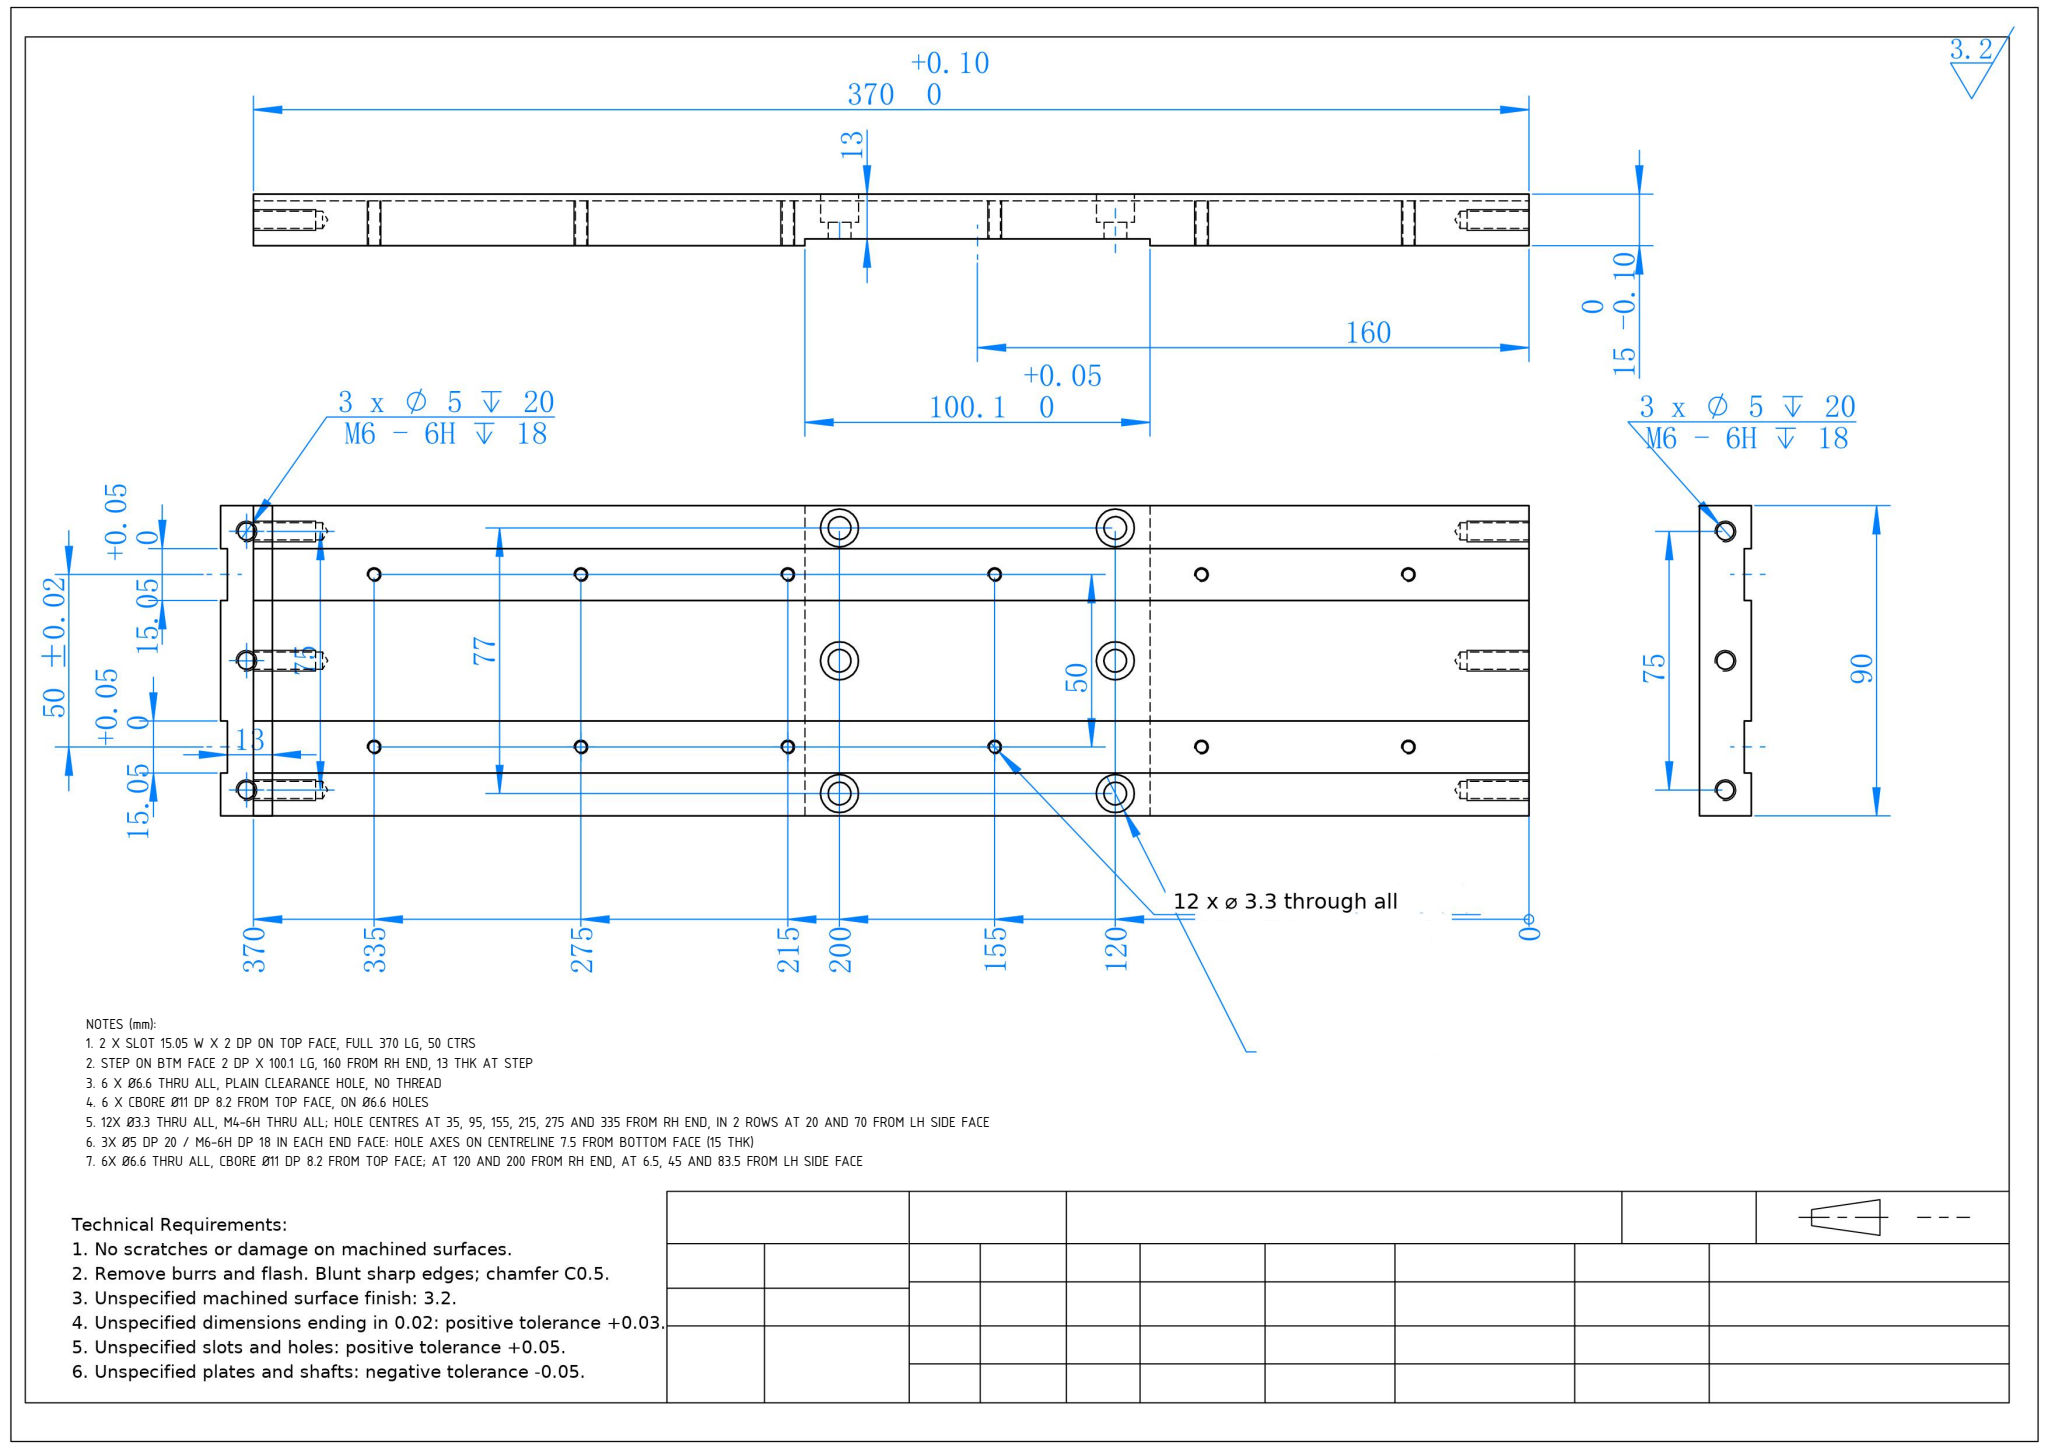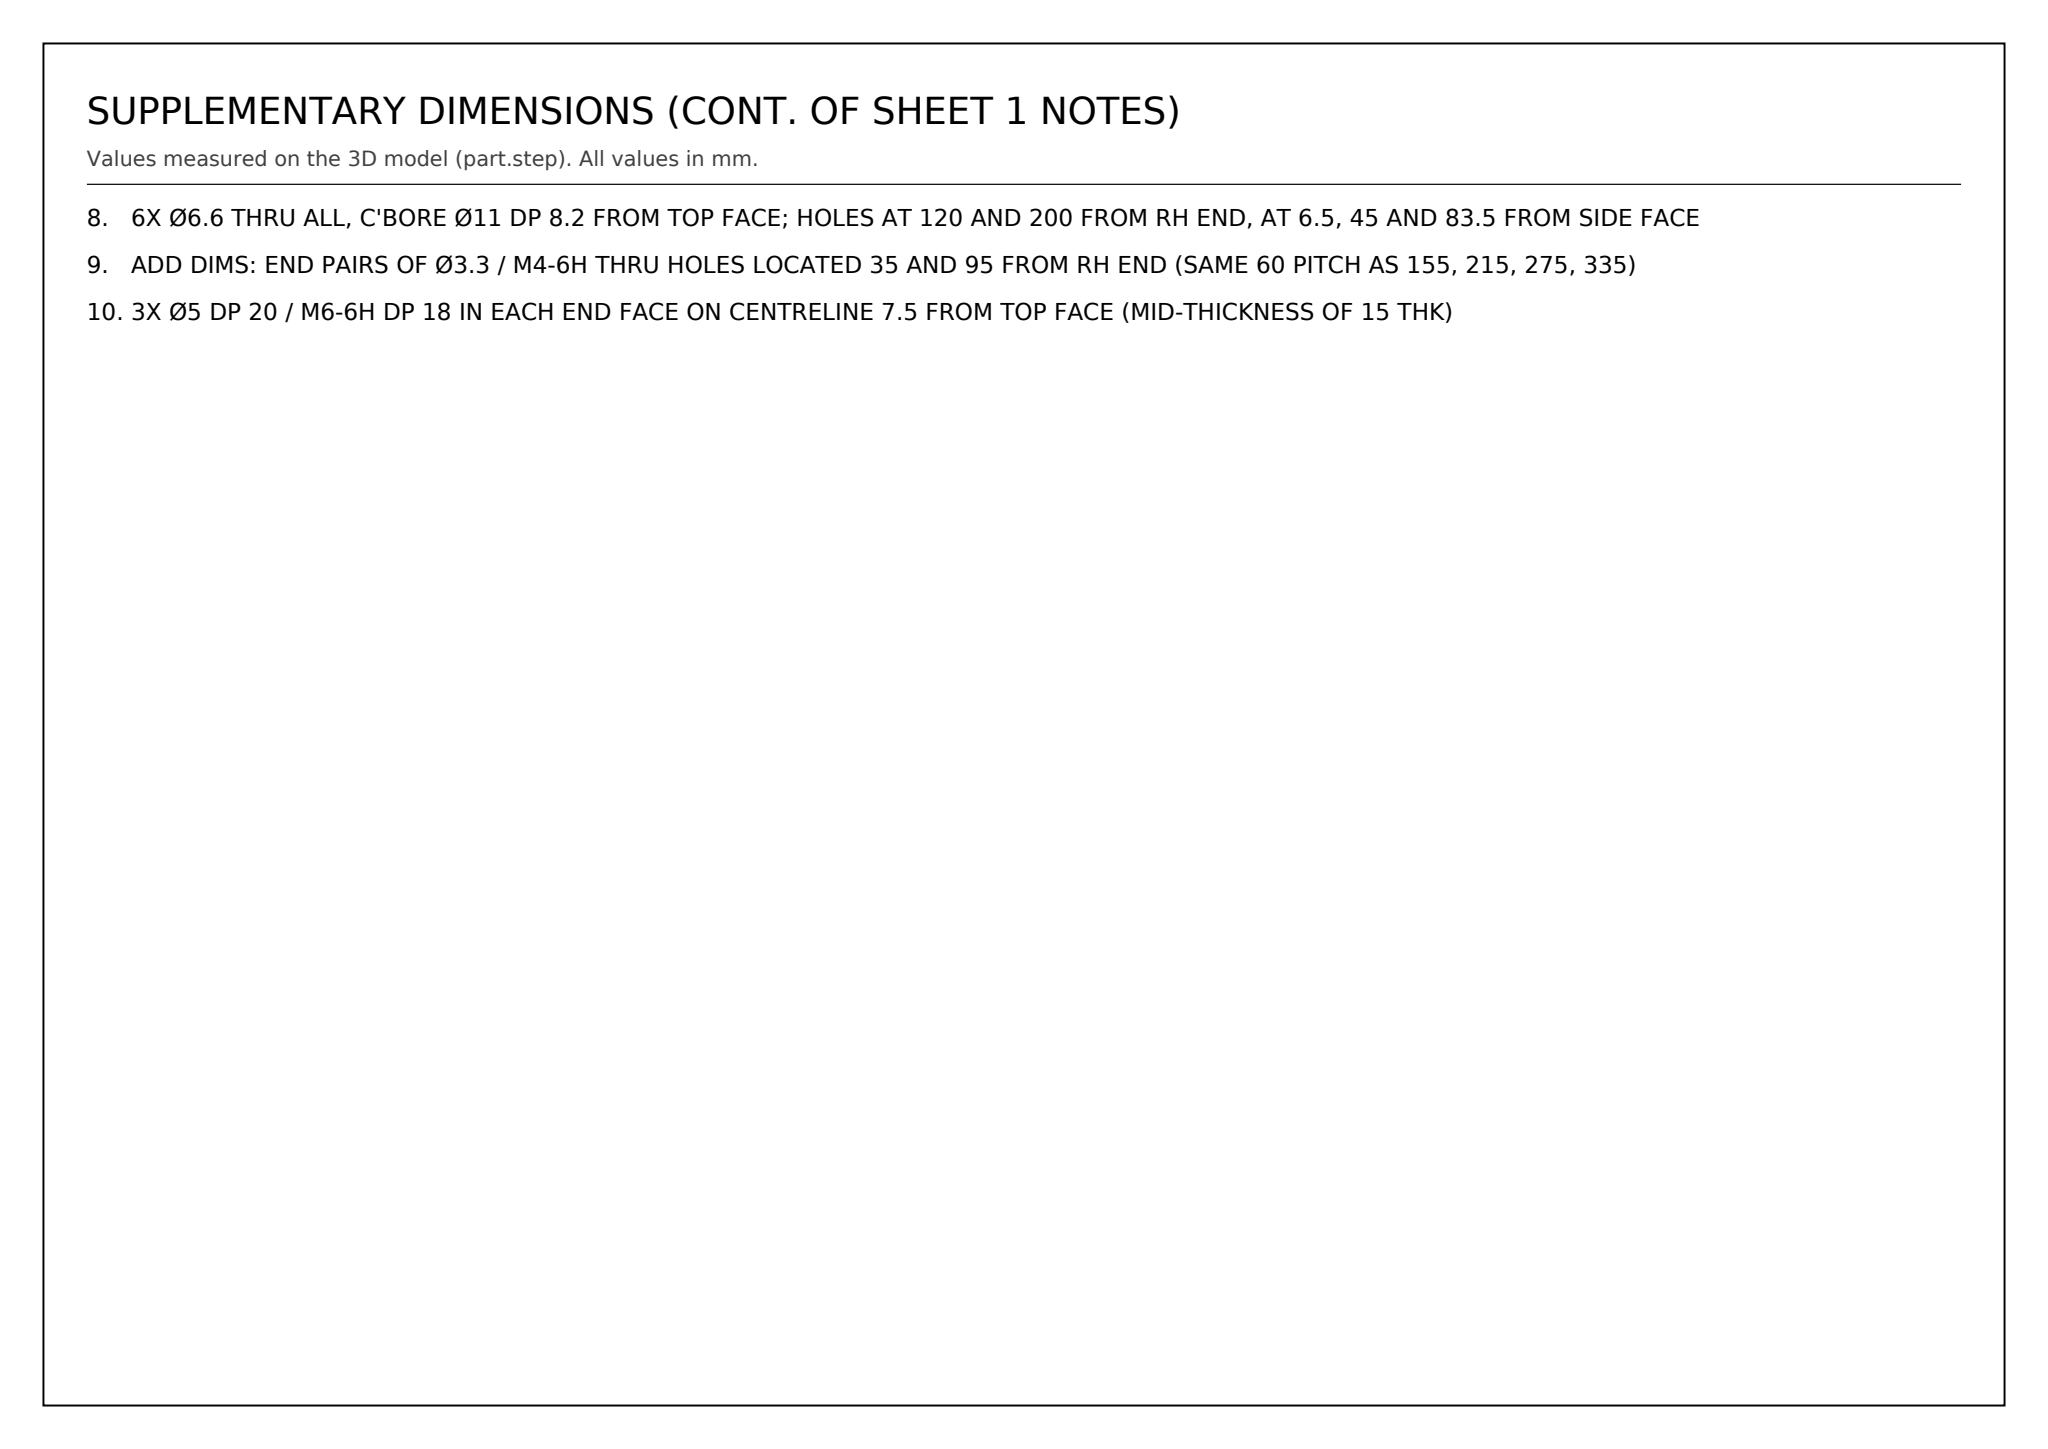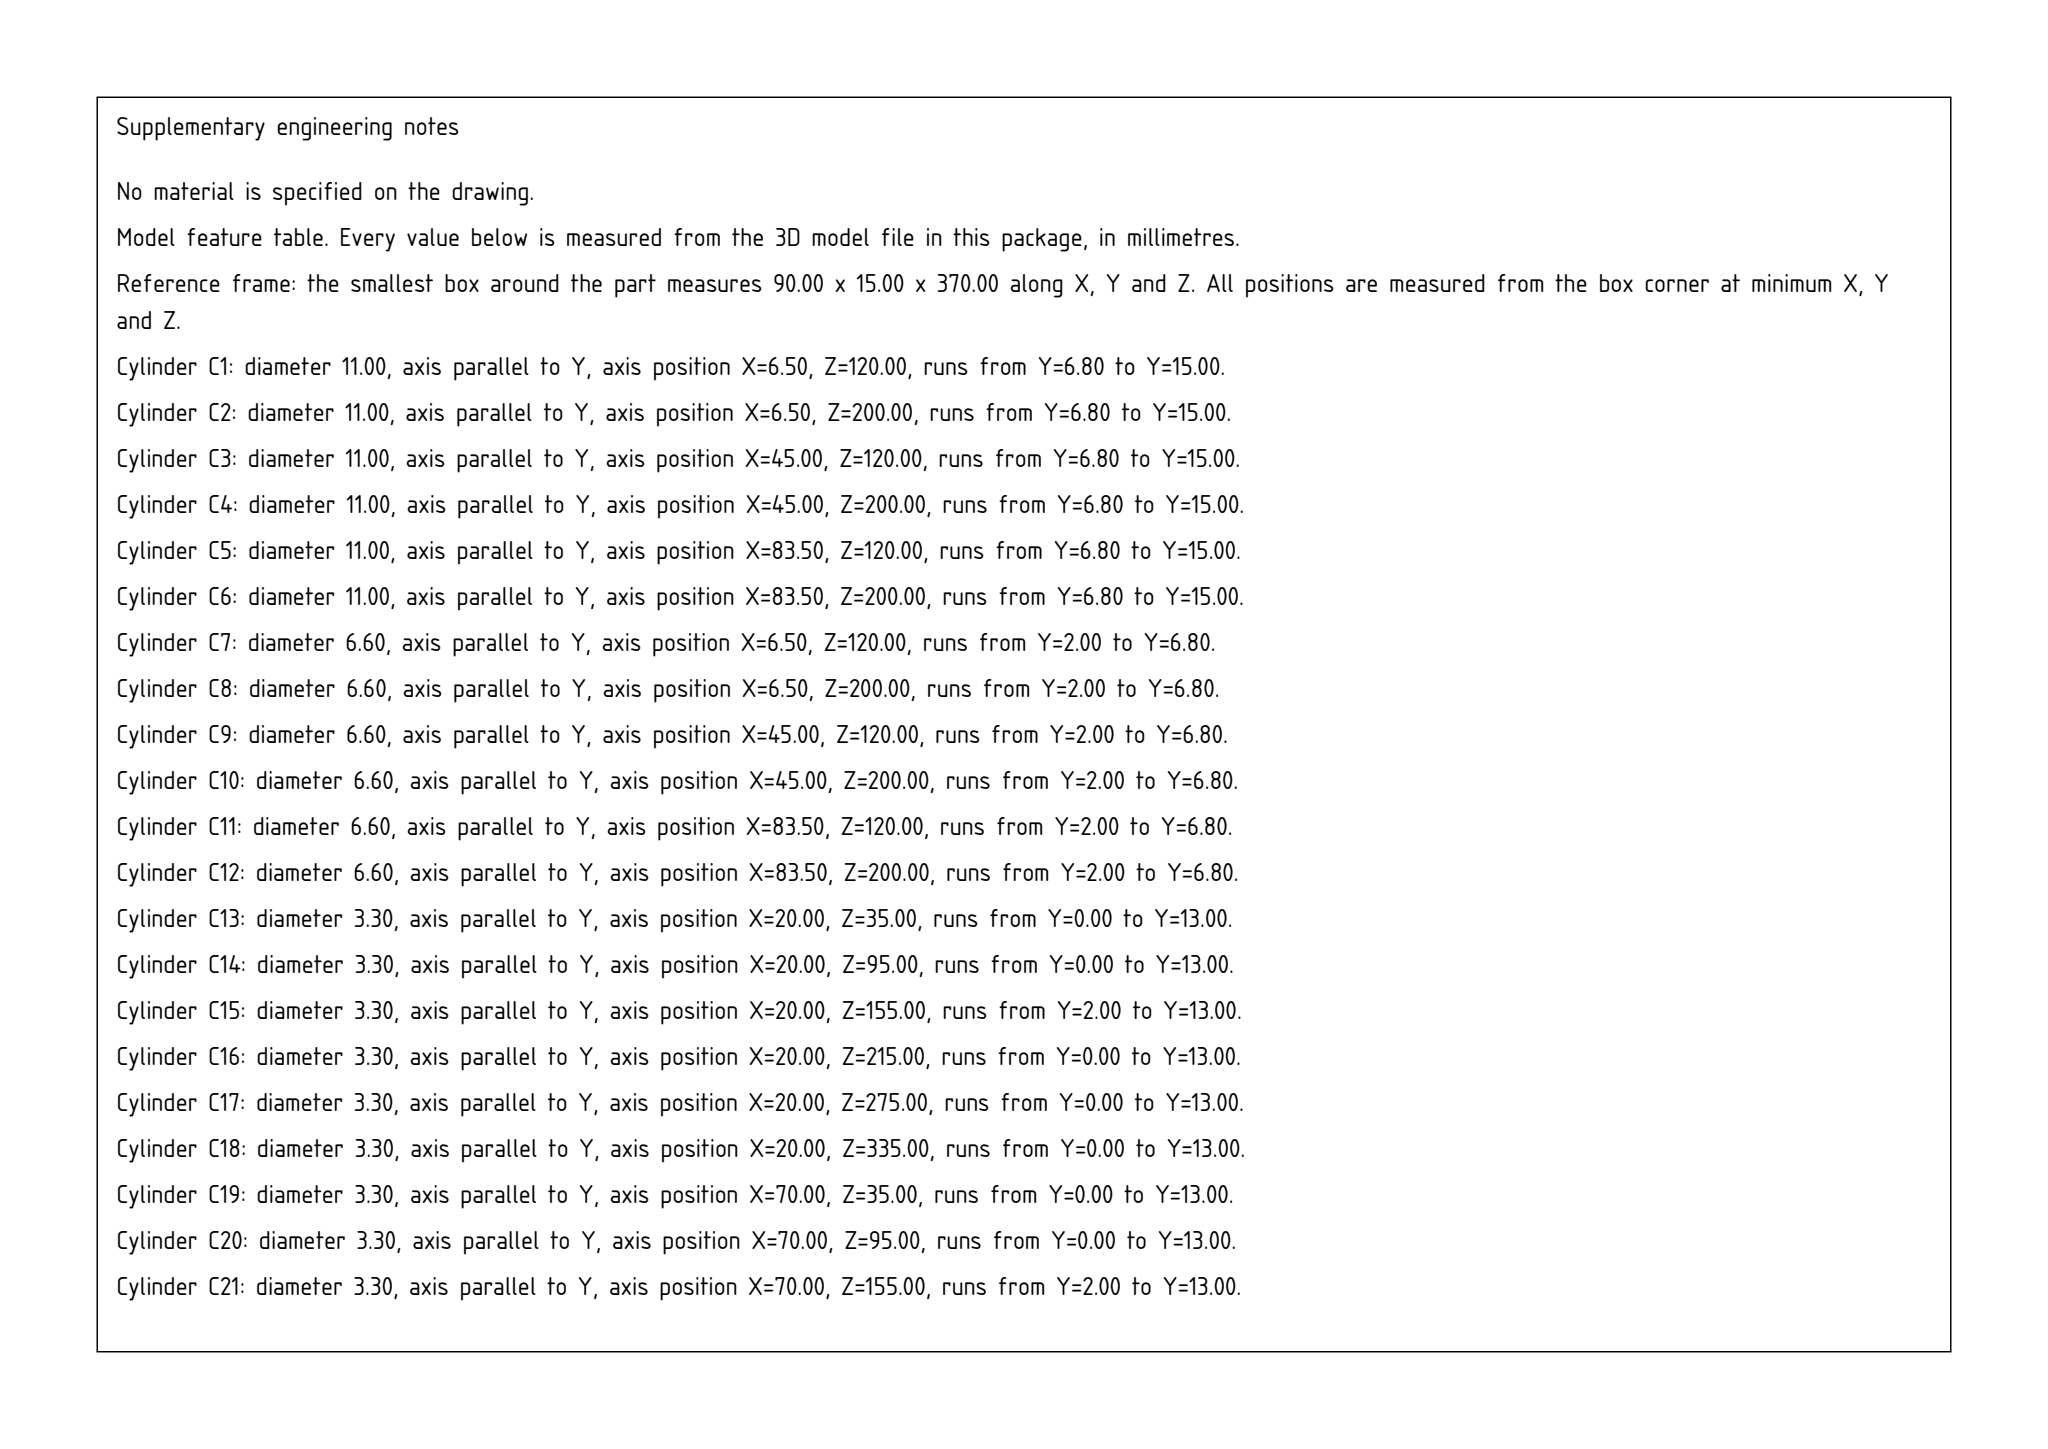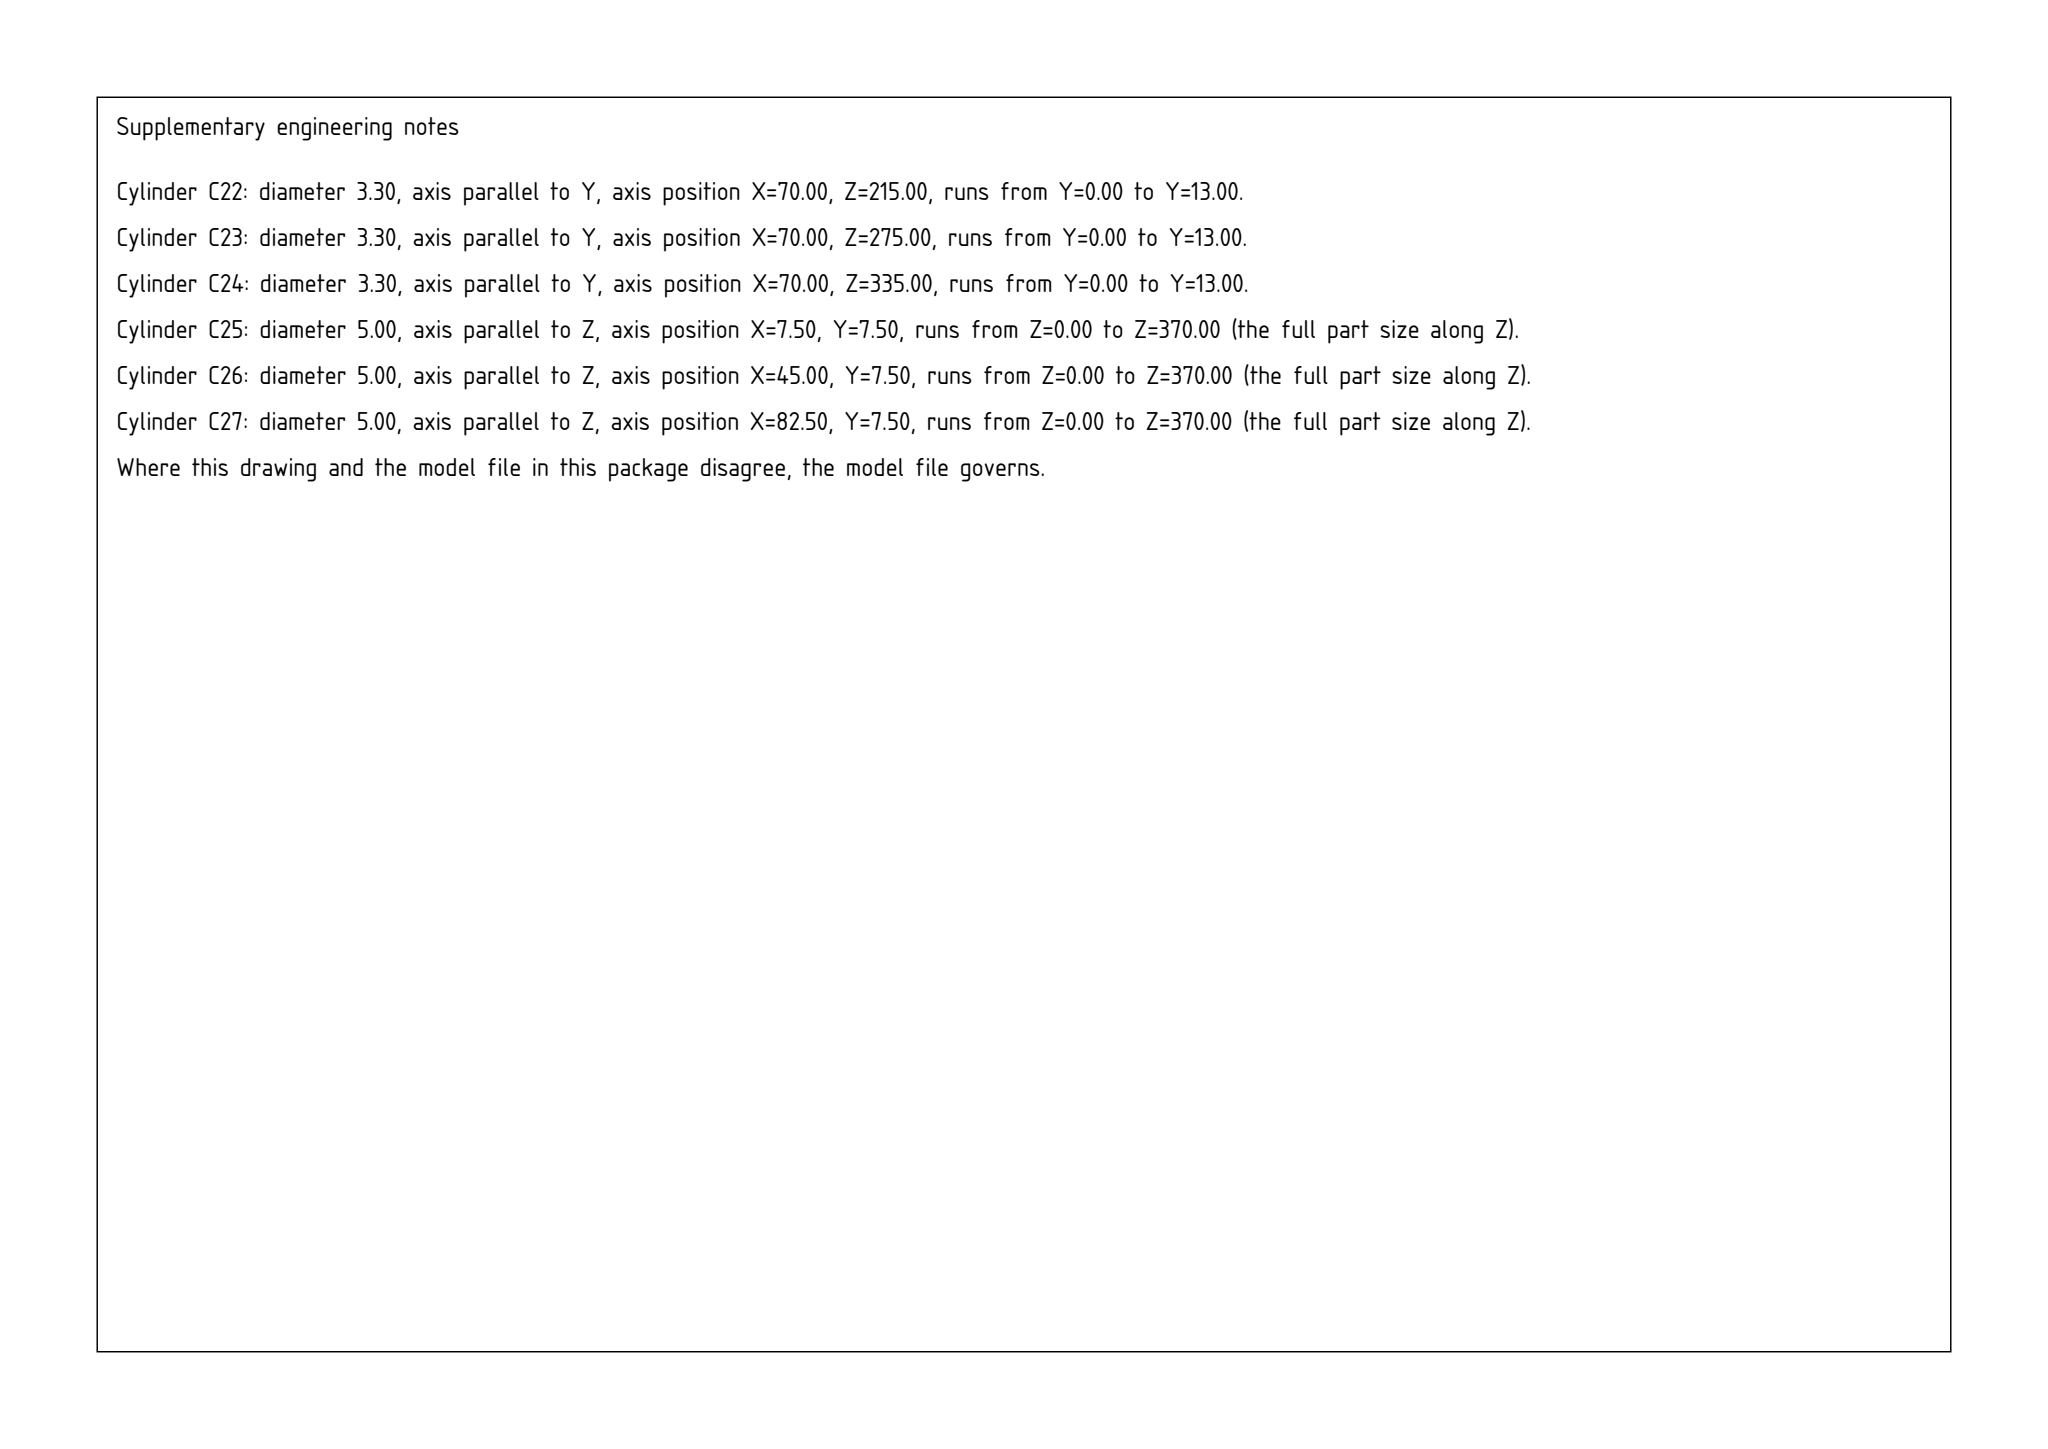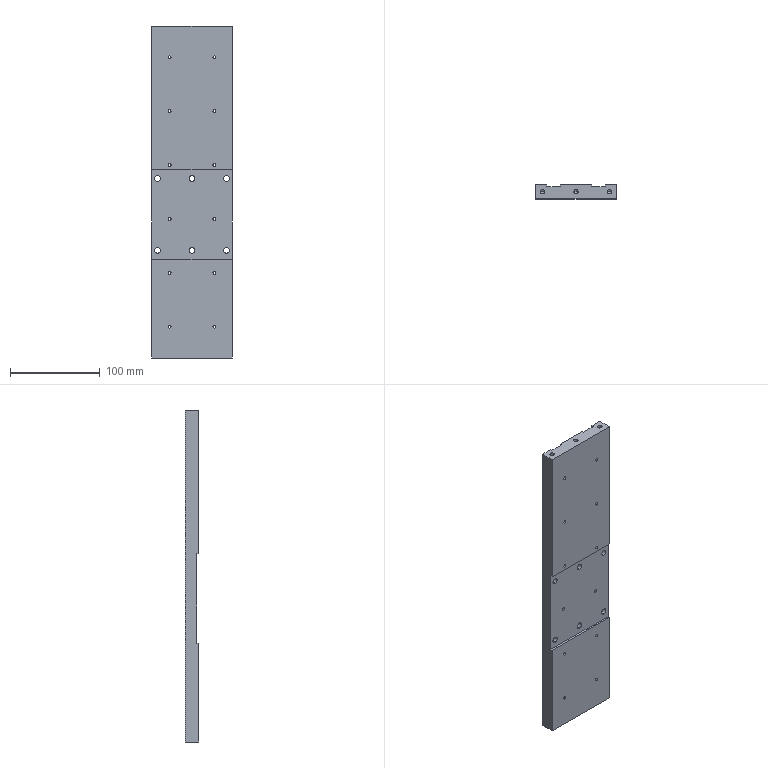Part | SolidWorks | mm | 1 solid | 96 faces | box 90 x 15 x 370 mm | volume 449832 mm3 | cylinder 60 | plane 24 | cone 12 | commonest cylinder face diameters 3.3 x24 11 x12 6.6 x12 5 x12
Drawing notes:
2 X SLOT 15.05 W X 2 DP ON TOP FACE, FULL 370 LG, 50 CTRS | from the solid: x planes 12.48/27.53 & 62.48/77.53 (w=15.05, CL 20.0 & 70.0); floor y=13 vs top y=15
STEP ON BTM FACE 2 DP X 100.1 LG, 160 FROM RH END, 13 THK AT STEP | from the solid: z planes 109.95 & 210.05 (100.1 lg), 370-210.05=160; floor y=2.0, thk 13
6 X Ø6.6 THRU ALL, PLAIN CLEARANCE HOLE, NO THREAD | from the solid: cyl Ø6.6 axis y len 4.8 at x=6.5/45/83.5, z=120 & 200 (6 plcs)
6 X CBORE Ø11 DP 8.2 FROM TOP FACE, ON Ø6.6 HOLES | from the solid: cyl Ø11 axis y len 8.2, floor y=6.8 (6 plcs) from top y=15
12X Ø3.3 THRU ALL, M4-6H THRU ALL; HOLE CENTRES AT 35, 95, 155, 215, 275 AND 335 FROM RH END, IN 2 ROWS AT 20 AND 70 FROM LH SIDE FACE | from the solid: cylinders dia 3.3 axis y at z=35, 95, 155, 215, 275, 335 and x=20.0 / 70.0
3X Ø5 DP 20 / M6-6H DP 18 IN EACH END FACE: HOLE AXES ON CENTRELINE 7.5 FROM BOTTOM FACE (15 THK) | from the solid: cylinders dia 5.0 axis z, pos_other_axes y=7.5, length 20.0
6X Ø6.6 THRU ALL, CBORE Ø11 DP 8.2 FROM TOP FACE; AT 120 AND 200 FROM RH END, AT 6.5, 45 AND 83.5 FROM LH SIDE FACE | from the solid: cylinders dia 6.6 (len 4.8) and dia 11.0 (len 8.2) axis y at z=120.0, 200.0 and x=6.5, 45.0, 83.5
6X Ø6.6 THRU ALL, C'BORE Ø11 DP 8.2 FROM TOP FACE; HOLES AT 120 AND 200 FROM RH END, AT 6.5, 45 AND 83.5 FROM SIDE FACE | from the solid: cylinders dia 6.6 axis y at (6.5/45/83.5, z=120 & 200) len 4.8 and dia 11.0 axis y same positions len 8.2
ADD DIMS: END PAIRS OF Ø3.3 / M4-6H THRU HOLES LOCATED 35 AND 95 FROM RH END (SAME 60 PITCH AS 155, 215, 275, 335) | from the solid: cylinders dia 3.3 axis y at z=35 and z=95, x=20.0 and 70.0
3X Ø5 DP 20 / M6-6H DP 18 IN EACH END FACE ON CENTRELINE 7.5 FROM TOP FACE (MID-THICKNESS OF 15 THK) | from the solid: cylinders dia 5.0 axis z at y=7.5 (x=7.5, 45.0, 82.5), length 20.0
build123d program:
from build123d import *

# Parameters (mm, degrees)
SKETCH1_W                                       = 90
SKETCH1_H                                       = 15
EXTRUDE1_DEPTH                                  = 185
SKETCH16_W                                      = 15.05
SKETCH16_H                                      = 370
CUT_EXTRUDE1_DEPTH                              = 2
SKETCH17_W                                      = 90
SKETCH17_H                                      = 100.1
CUT_EXTRUDE2_DEPTH                              = 2
M6_TAPPED_HOLE1_D                               = 5
M6_TAPPED_HOLE1_DEPTH                           = 20
M6_TAPPED_HOLE1_TIP                             = 1.502
M6_TAPPED_HOLE2_D                               = 5
M6_TAPPED_HOLE2_DEPTH                           = 20
M6_TAPPED_HOLE2_TIP                             = 1.502
M6_HEX_SOCKET_HEAD_CAP_SCREW_CBORE1_D           = 6.6
M6_HEX_SOCKET_HEAD_CAP_SCREW_CBORE1_CBORE_D     = 11
M6_HEX_SOCKET_HEAD_CAP_SCREW_CBORE1_CBORE_DEPTH = 8.2
M4_TAPPED_HOLE8_D                               = 3.3


with BuildPart() as part:
    # Sketch1 → Extrude1 (new, symmetric)
    with BuildSketch(Plane.XY):
        Rectangle(SKETCH1_W, SKETCH1_H)
    extrude(amount=EXTRUDE1_DEPTH, both=True)

    # Sketch16 → Cut-Extrude1 (cut)
    with BuildSketch(Plane(origin=(0, 7.5, 0), x_dir=(1, 0, 0), z_dir=(0, 1, 0))):
        with Locations((25, 0)):
            Rectangle(SKETCH16_W, SKETCH16_H)
        with Locations((-25, 0)):
            Rectangle(SKETCH16_W, SKETCH16_H)
    extrude(amount=-CUT_EXTRUDE1_DEPTH, mode=Mode.SUBTRACT)

    # Sketch17 → Cut-Extrude2 (cut)
    with BuildSketch(Plane(origin=(0, -7.5, 0), x_dir=(-1, 0, 0), z_dir=(0, -1, 0))):
        with Locations((0, 25)):
            Rectangle(SKETCH17_W, SKETCH17_H)
    extrude(amount=-CUT_EXTRUDE2_DEPTH, mode=Mode.SUBTRACT)

    # M6 Tapped Hole1
    with Locations(Plane(origin=(0, 0, -185), x_dir=(-1, 0, 0), z_dir=(0, 0, -1))):
        with Locations((-37.5, 0), (0, 0), (37.5, 0)):
            Hole(M6_TAPPED_HOLE1_D / 2, depth=M6_TAPPED_HOLE1_DEPTH)
            with Locations((0, 0, -(M6_TAPPED_HOLE1_DEPTH + M6_TAPPED_HOLE1_TIP / 2))):  # 118° drill point
                Cone(0, M6_TAPPED_HOLE1_D / 2, M6_TAPPED_HOLE1_TIP, mode=Mode.SUBTRACT)

    # M6 Tapped Hole2
    with Locations(Plane.XY.offset(185)):
        with Locations((-37.5, 0), (37.5, 0), (0, 0)):
            Hole(M6_TAPPED_HOLE2_D / 2, depth=M6_TAPPED_HOLE2_DEPTH)
            with Locations((0, 0, -(M6_TAPPED_HOLE2_DEPTH + M6_TAPPED_HOLE2_TIP / 2))):  # 118° drill point
                Cone(0, M6_TAPPED_HOLE2_D / 2, M6_TAPPED_HOLE2_TIP, mode=Mode.SUBTRACT)

    # M6 Hex Socket Head Cap Screw CBORE1 (through all)
    with Locations(Plane(origin=(0, 7.5, 0), x_dir=(-1, 0, 0), z_dir=(0, 1, 0))):
        with Locations((-38.5, -65), (38.5, -65), (38.5, 15), (-38.5, 15), (0, -65), (0, 15)):
            CounterBoreHole(M6_HEX_SOCKET_HEAD_CAP_SCREW_CBORE1_D / 2, M6_HEX_SOCKET_HEAD_CAP_SCREW_CBORE1_CBORE_D / 2, M6_HEX_SOCKET_HEAD_CAP_SCREW_CBORE1_CBORE_DEPTH)

    # M4 Tapped Hole8 (through all)
    with Locations(Plane(origin=(0, 7.5, 0), x_dir=(-1, 0, 0), z_dir=(0, 1, 0))):
        with Locations((-25, -30), (-25, 90), (-25, 150), (-25, 30), (25, 30), (25, 150), (25, 90), (25, -30), (25, -90), (-25, -90), (-25, -150), (25, -150)):
            Hole(M4_TAPPED_HOLE8_D / 2)


solid = part.part